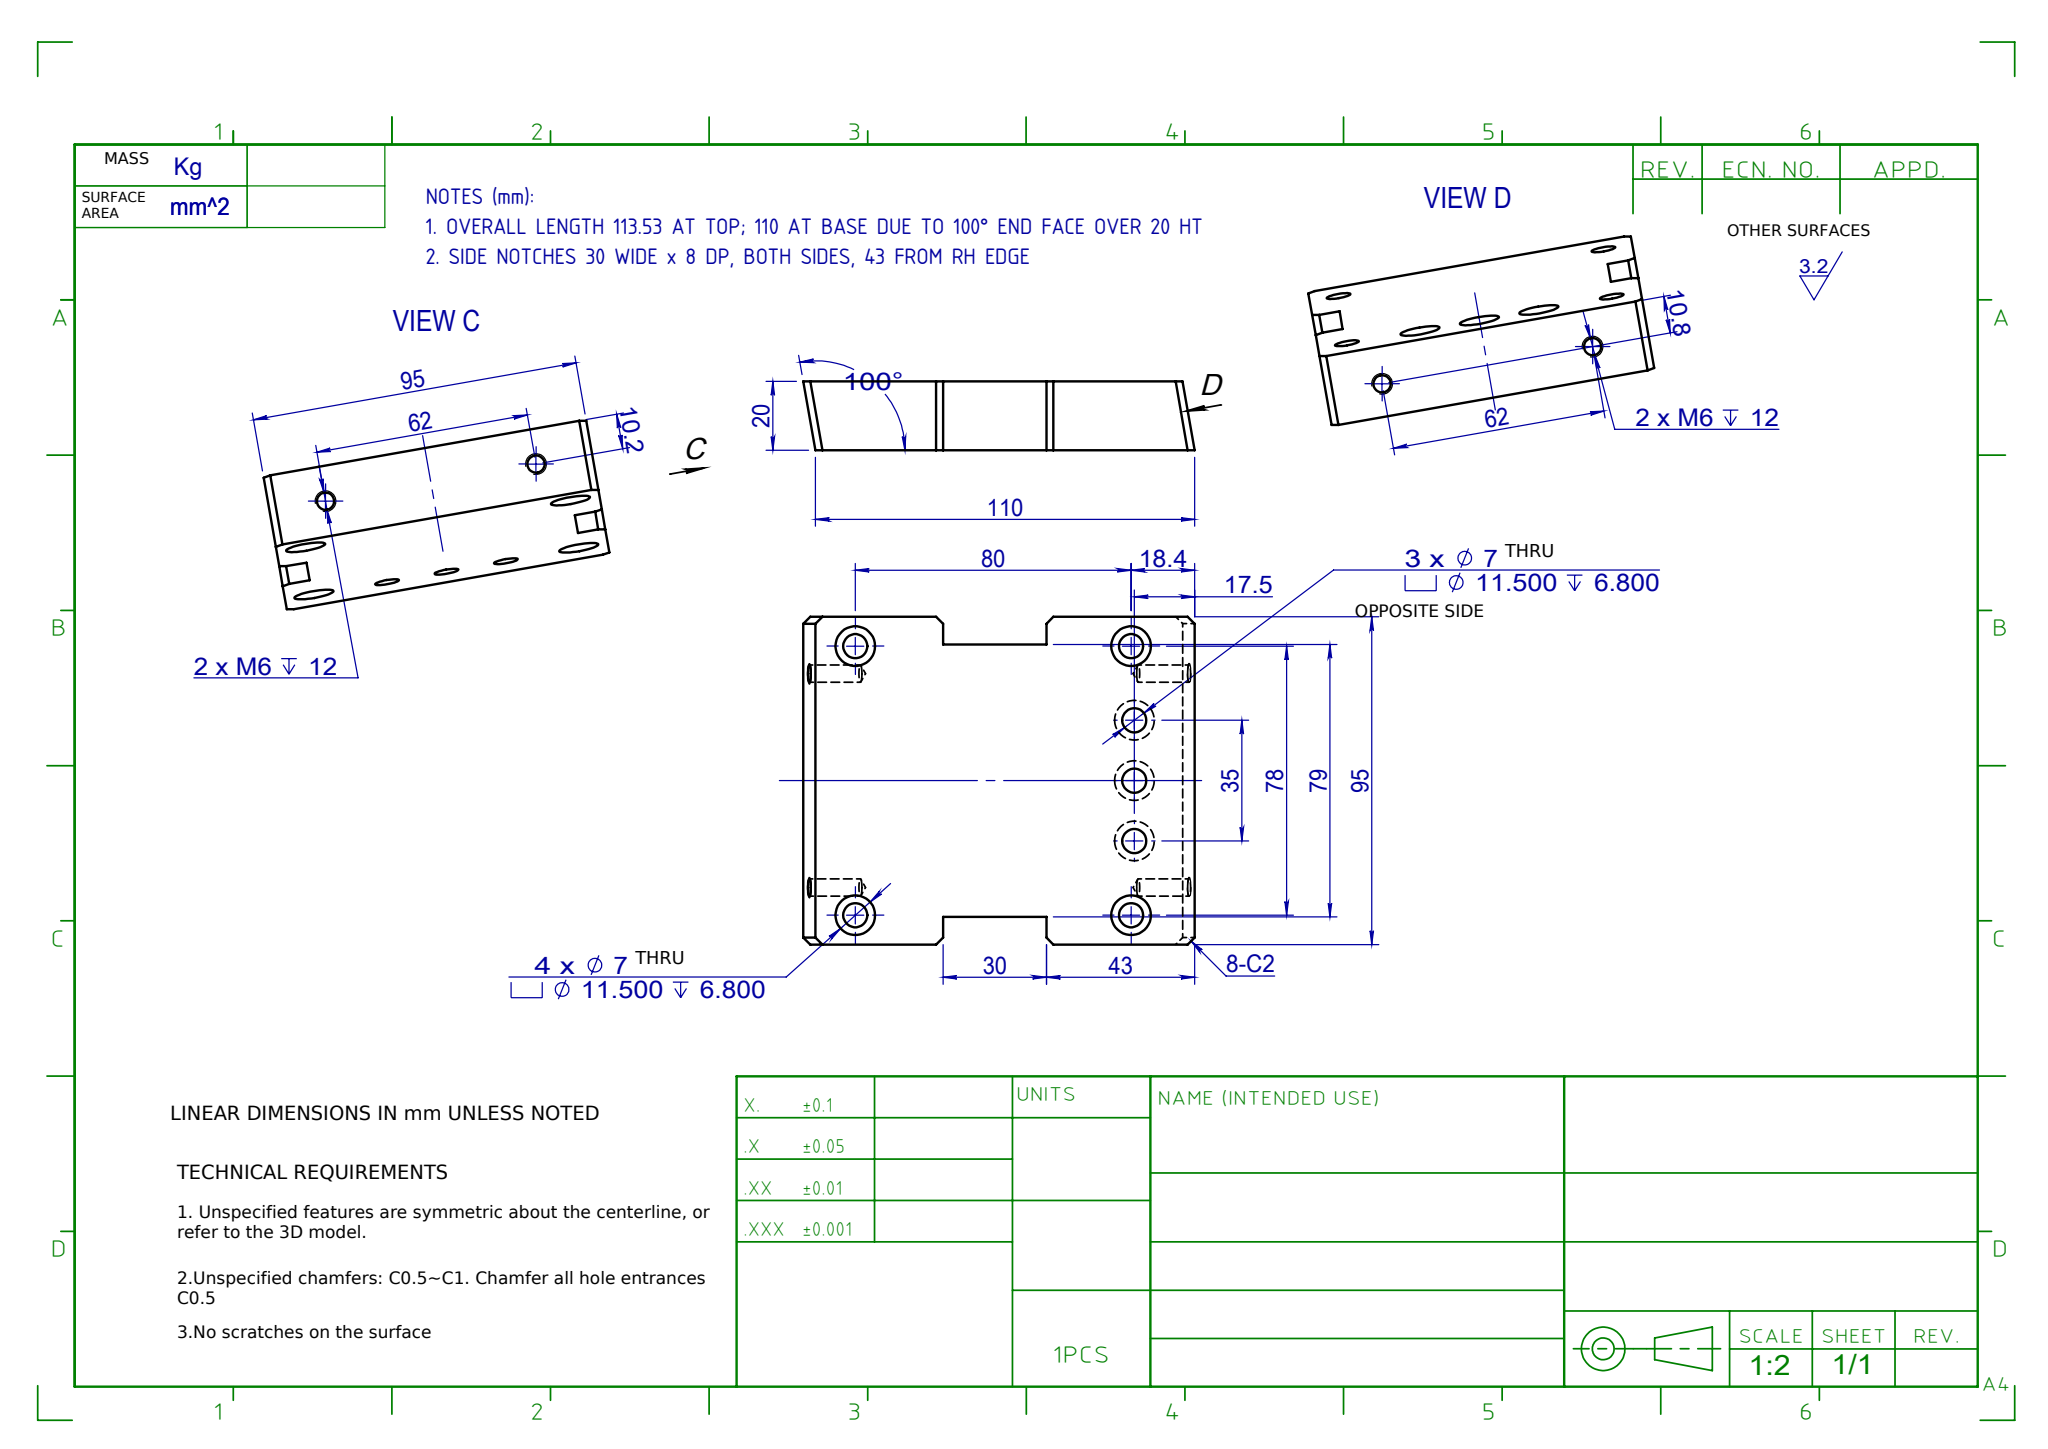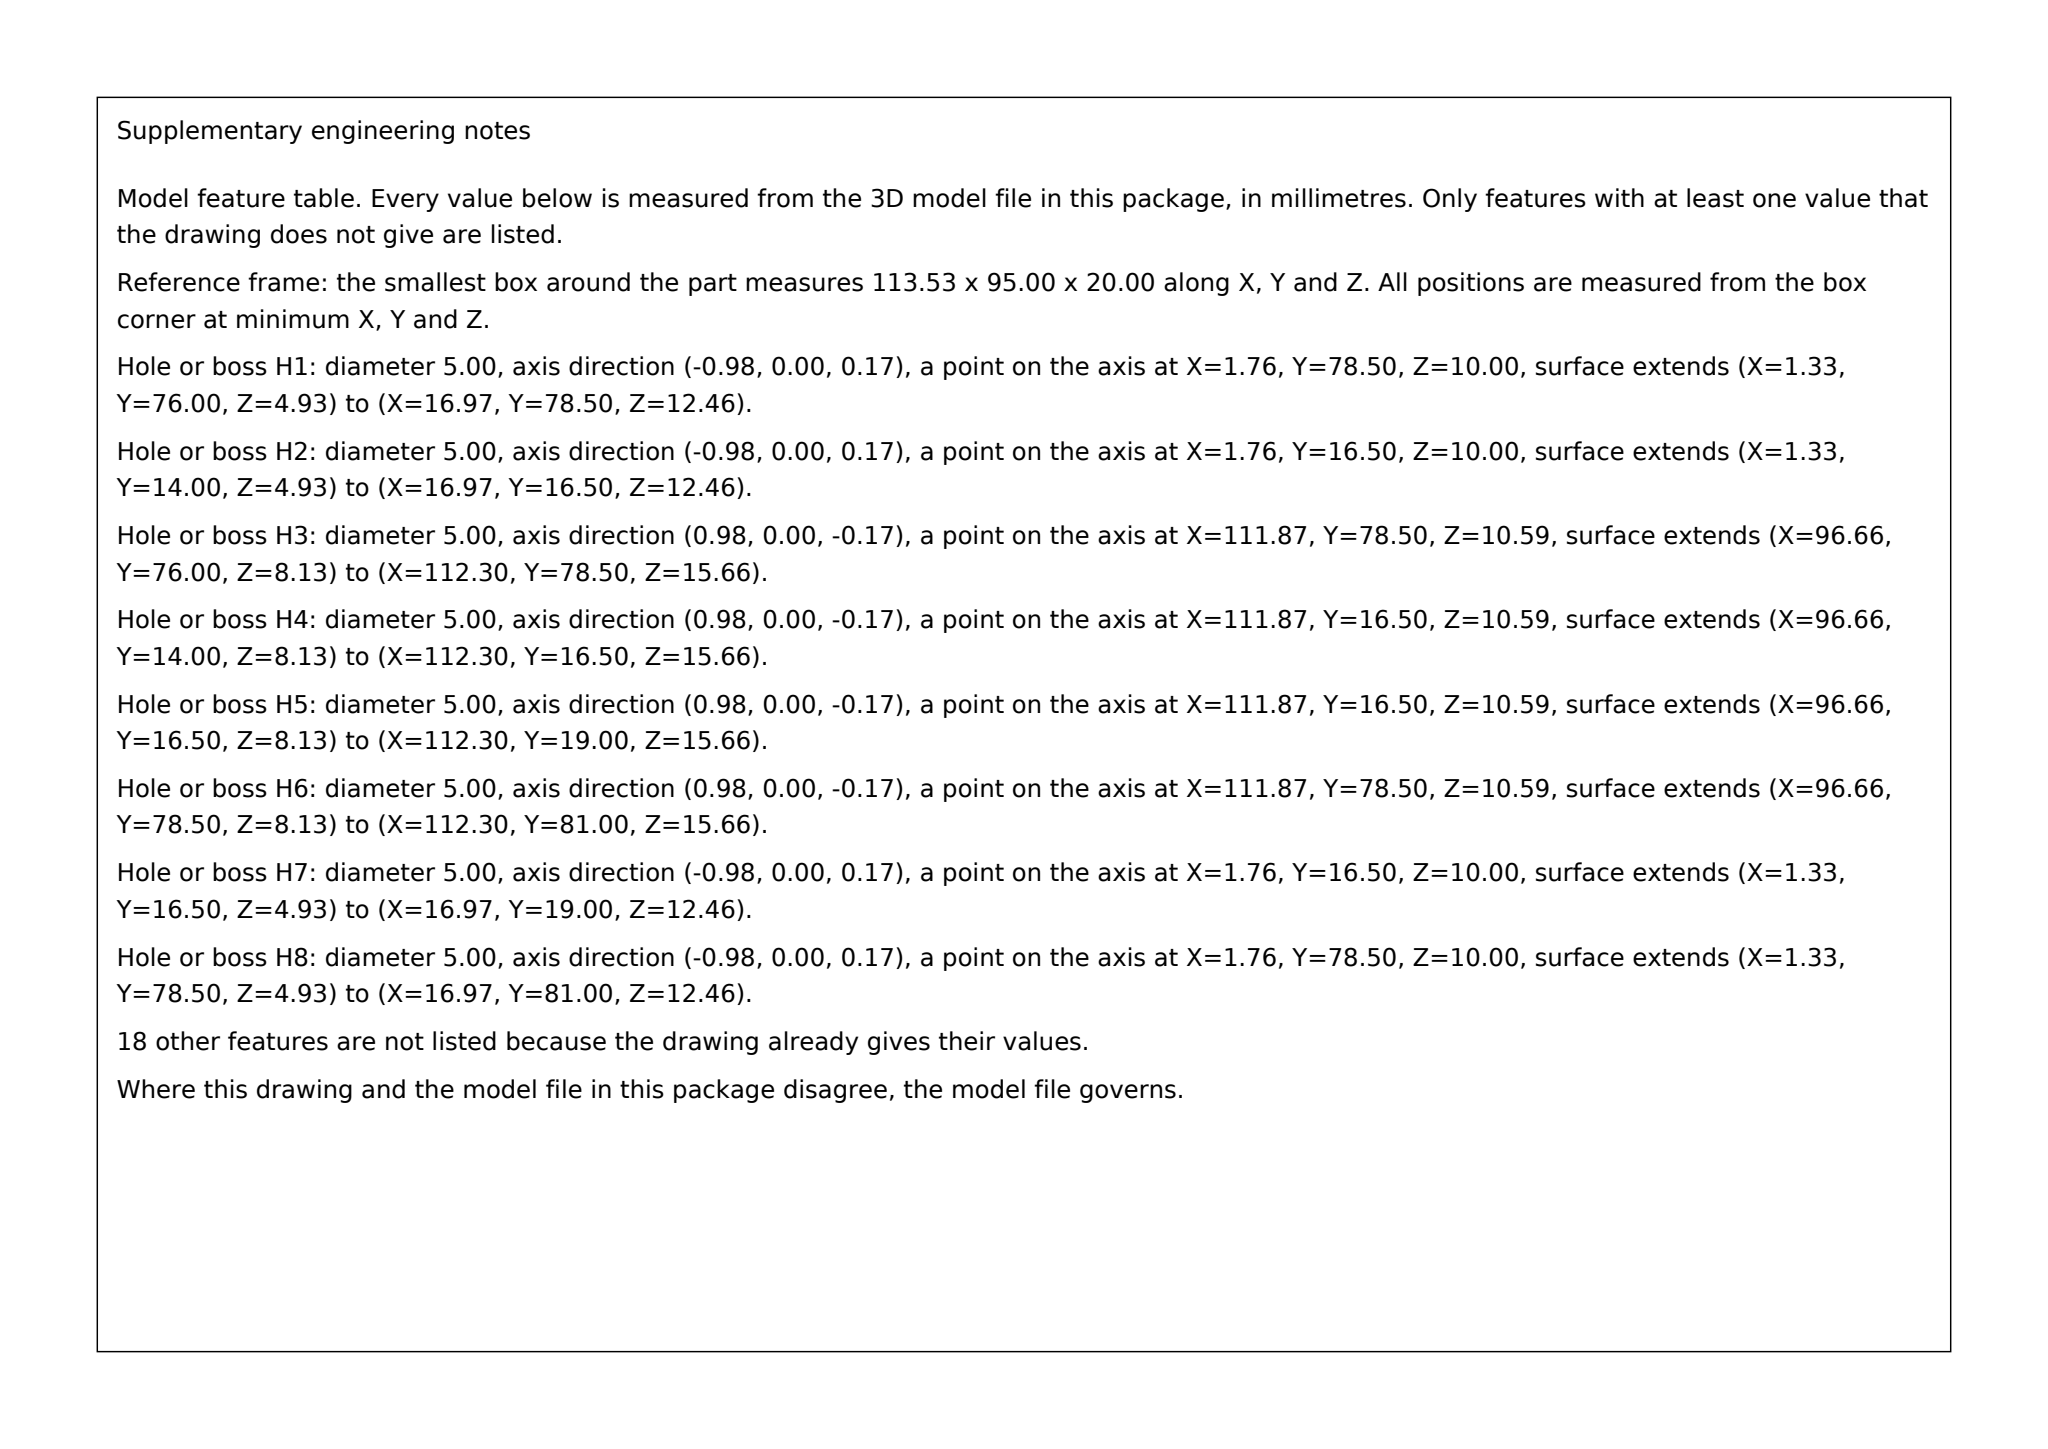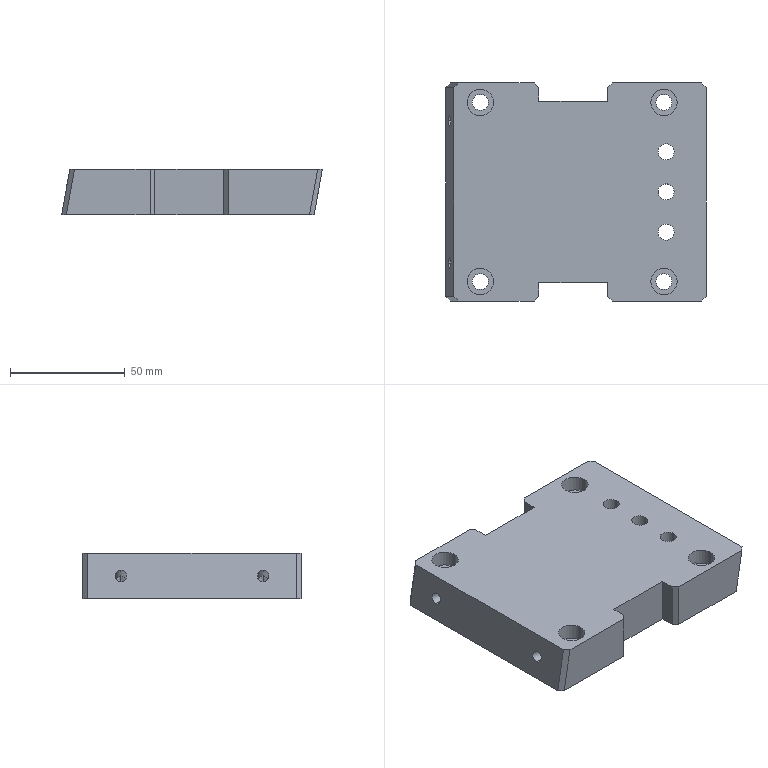Part | SolidWorks | mm | 1 solid | 73 faces | box 113.53 x 95 x 20 mm | volume 189360 mm3 | cylinder 36 | plane 29 | cone 8 | commonest cylinder face diameters 11.5 x14 7 x14 5 x8
Drawing notes:
OVERALL LENGTH 113.53 AT TOP; 110 AT BASE DUE TO 100° END FACE OVER 20 HT | from the solid: bbox_xyz x=113.527 vs 110 dim; 20*tan10=3.527 offset over full 20 thickness
SIDE NOTCHES 30 WIDE x 8 DP, BOTH SIDES, 43 FROM RH EDGE | from the solid: Planes x=40.53 & x=70.53 (width 30); y=8.0 and y=87.0 vs y=0/95 faces give 8 deep; 113.527-70.53=43
build123d program:
from build123d import *

# Parameters (mm, degrees)
SKETCH1_2_W                                          = 110
SKETCH1_2_H                                          = 95
SKETCH3_2_W                                          = 30
SKETCH3_2_H                                          = 8
CUT_EXTRUDE1_DEPTH                                   = 78.985
M6_TAPPED_HOLE1_D                                    = 5
M6_TAPPED_HOLE1_DEPTH                                = 15
M6_TAPPED_HOLE1_TIP                                  = 1.502
M6_TAPPED_HOLE2_D                                    = 5
M6_TAPPED_HOLE2_DEPTH                                = 15
M6_TAPPED_HOLE2_TIP                                  = 1.502
CBORE_FOR_M6_HEXAGON_SOCKET_HEAD_CAP_SCR_D           = 7
CBORE_FOR_M6_HEXAGON_SOCKET_HEAD_CAP_SCR_CBORE_D     = 11.5
CBORE_FOR_M6_HEXAGON_SOCKET_HEAD_CAP_SCR_CBORE_DEPTH = 6.8
CBORE_FOR_M6_HEXAGON_SOCKET_HEAD_CAP_2_D             = 7
CBORE_FOR_M6_HEXAGON_SOCKET_HEAD_CAP_2_CBORE_D       = 11.5
CBORE_FOR_M6_HEXAGON_SOCKET_HEAD_CAP_2_CBORE_DEPTH   = 6.8
CHAMFER1_SIZE                                        = 2


with BuildPart() as part:
    # Sweep1: sweep along a path in Sketch2_2
    with BuildLine(Plane(origin=(0, 0, 0), x_dir=(1, 0, 0), z_dir=(0, 1, 0))) as sweep1_path:
        Line((0, 0), (-3.527, 20))
    # Sketch1_2 → Sweep1 (sweep)
    with BuildSketch(Plane.XY):
        Rectangle(SKETCH1_2_W, SKETCH1_2_H)
    sweep(path=sweep1_path.line)

    # Sketch3_2 → Cut-Extrude1 (cut, through all)
    with BuildSketch(Plane.XY):
        with Locations((-3, 43.5)):
            Rectangle(SKETCH3_2_W, SKETCH3_2_H)
        with Locations((-3, -43.5)):
            Rectangle(SKETCH3_2_W, SKETCH3_2_H)
    extrude(amount=-CUT_EXTRUDE1_DEPTH, mode=Mode.SUBTRACT)

    # M6 Tapped Hole1
    with Locations(Plane(origin=(53.342, 0, -9.406), x_dir=(-0.1736, 0, -0.9848), z_dir=(0.9848, 0, -0.1736))):
        with Locations((0, 31), (0, -31)):
            Hole(M6_TAPPED_HOLE1_D / 2, depth=M6_TAPPED_HOLE1_DEPTH)
            with Locations((0, 0, -(M6_TAPPED_HOLE1_DEPTH + M6_TAPPED_HOLE1_TIP / 2))):  # 118° drill point
                Cone(0, M6_TAPPED_HOLE1_D / 2, M6_TAPPED_HOLE1_TIP, mode=Mode.SUBTRACT)

    # M6 Tapped Hole2
    with Locations(Plane(origin=(-53.342, 0, 9.406), x_dir=(0.1736, 0, 0.9848), z_dir=(-0.9848, 0, 0.1736))):
        with Locations((-19.705, 31), (-19.705, -31)):
            Hole(M6_TAPPED_HOLE2_D / 2, depth=M6_TAPPED_HOLE2_DEPTH)
            with Locations((0, 0, -(M6_TAPPED_HOLE2_DEPTH + M6_TAPPED_HOLE2_TIP / 2))):  # 118° drill point
                Cone(0, M6_TAPPED_HOLE2_D / 2, M6_TAPPED_HOLE2_TIP, mode=Mode.SUBTRACT)

    # CBORE for M6 Hexagon socket head cap scr (through all)
    with Locations(Plane(origin=(0, 0, -20), x_dir=(-1, 0, 0), z_dir=(0, 0, -1))):
        with Locations((-37.473, 17.5), (-37.473, 0), (-37.473, -17.5)):
            CounterBoreHole(CBORE_FOR_M6_HEXAGON_SOCKET_HEAD_CAP_SCR_D / 2, CBORE_FOR_M6_HEXAGON_SOCKET_HEAD_CAP_SCR_CBORE_D / 2, CBORE_FOR_M6_HEXAGON_SOCKET_HEAD_CAP_SCR_CBORE_DEPTH)

    # CBORE for M6 Hexagon socket head cap 2 (through all)
    with Locations(Plane.XY):
        with Locations((36.551, -39), (36.551, 39), (-43.449, 39), (-43.449, -39)):
            CounterBoreHole(CBORE_FOR_M6_HEXAGON_SOCKET_HEAD_CAP_2_D / 2, CBORE_FOR_M6_HEXAGON_SOCKET_HEAD_CAP_2_CBORE_D / 2, CBORE_FOR_M6_HEXAGON_SOCKET_HEAD_CAP_2_CBORE_DEPTH)

    # Chamfer1
    chamfer1_edges = [part.edges().sort_by_distance(p)[0] for p in [
        (12, 47.5, -10),
        (-18, 47.5, -10),
        (12, -47.5, -10),
        (-18, -47.5, -10),
        (-56.763, 47.5, -10),
        (53.237, 47.5, -10),
        (53.237, -47.5, -10),
        (-56.763, -47.5, -10),
    ]]
    chamfer(chamfer1_edges, length=CHAMFER1_SIZE)


solid = part.part